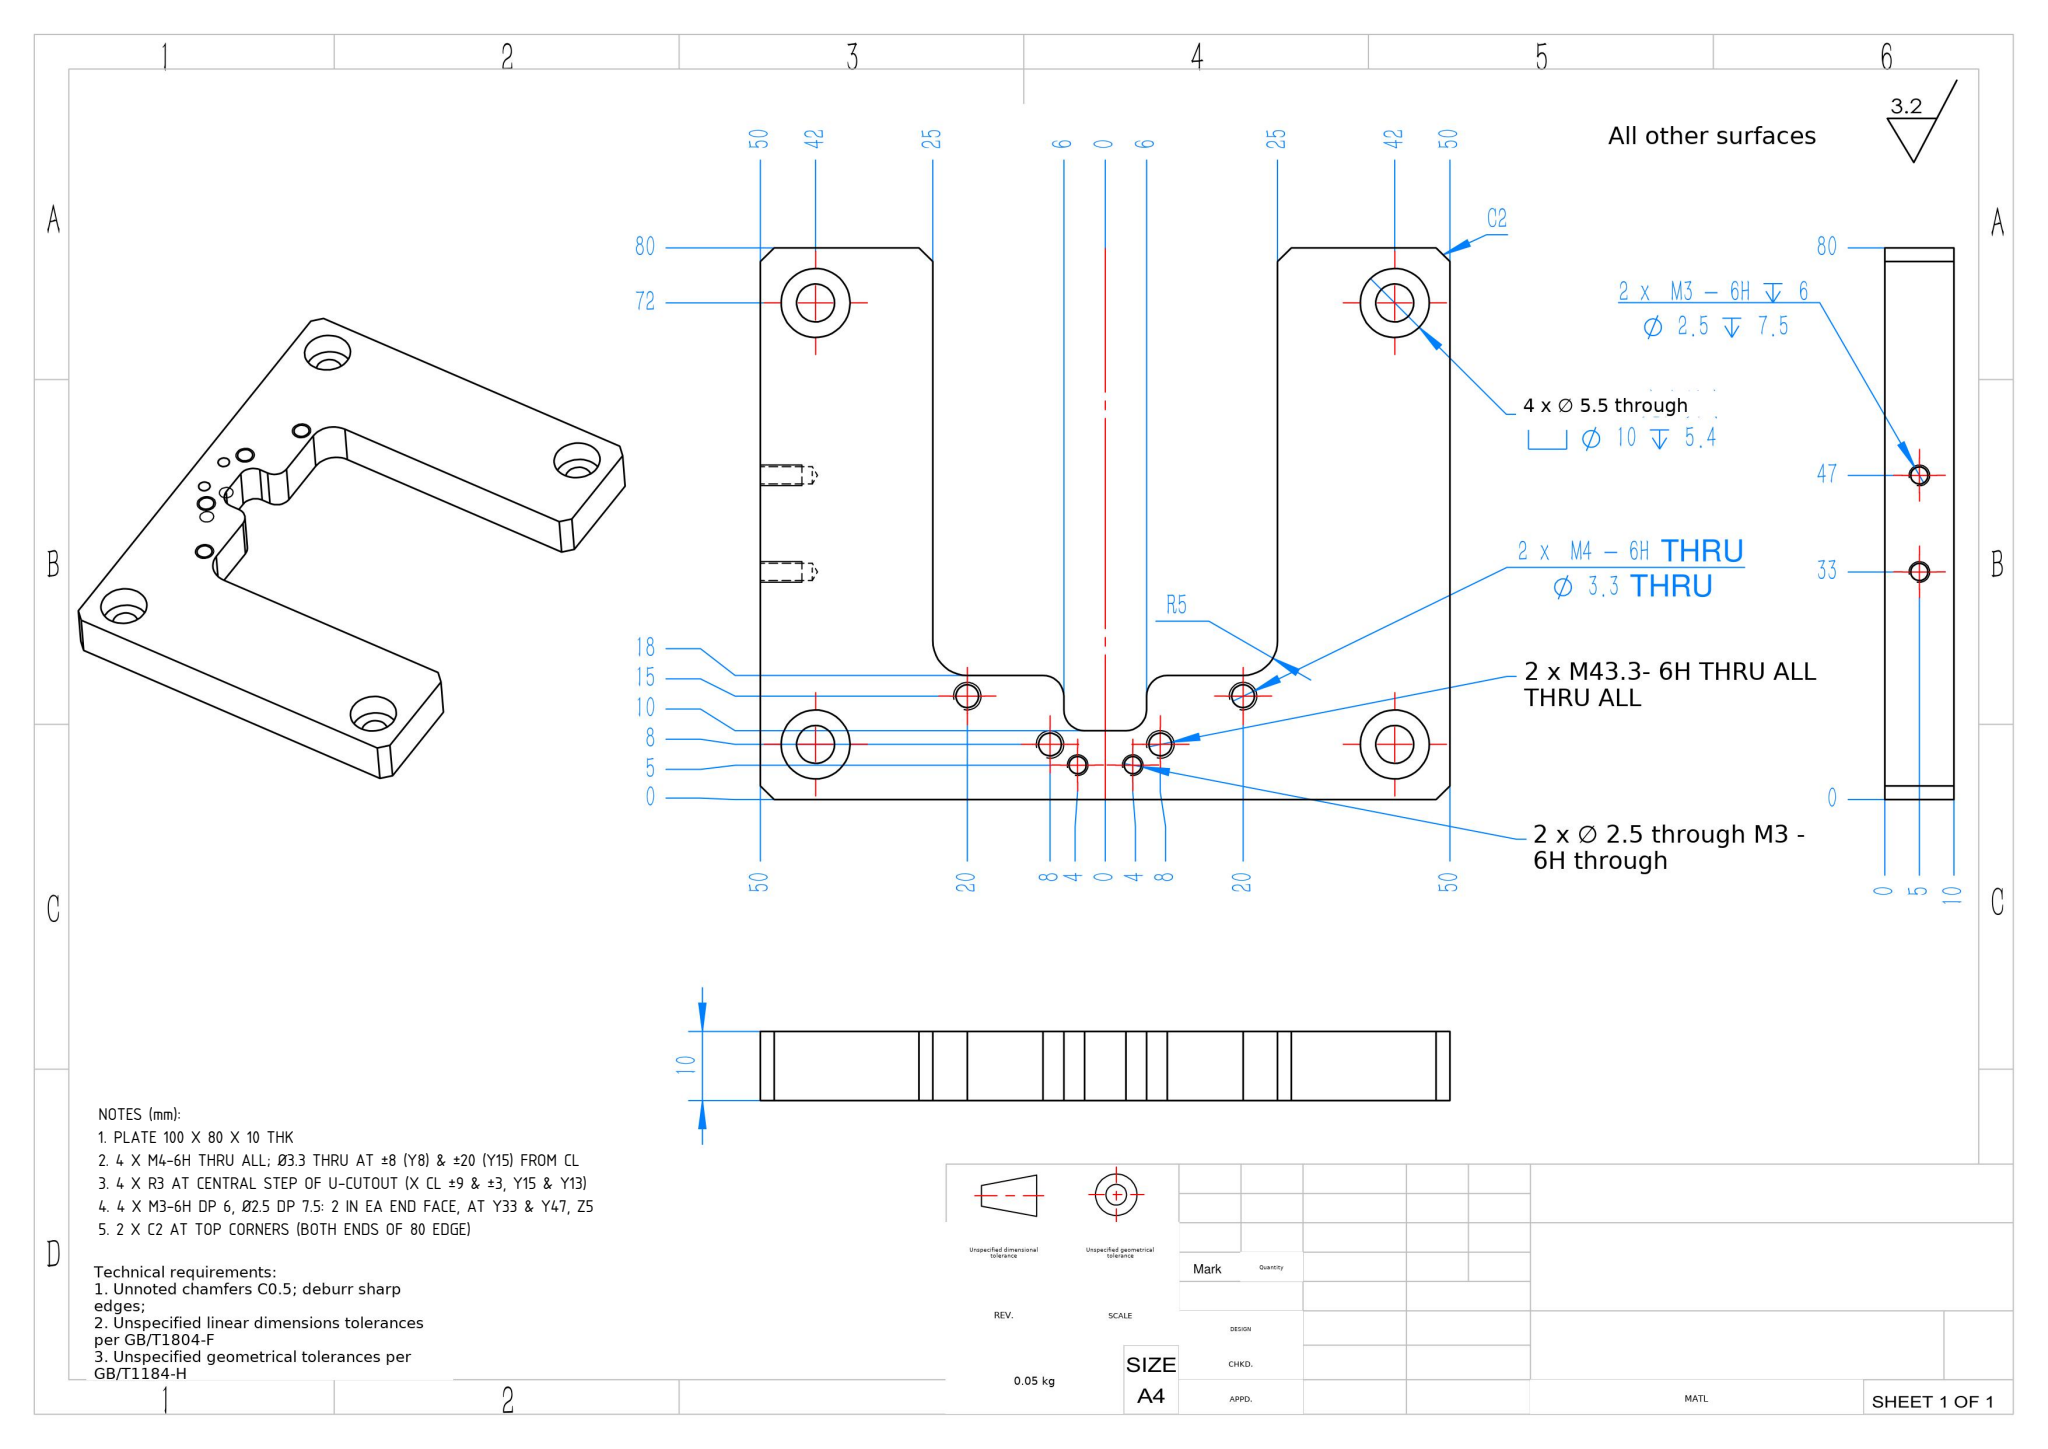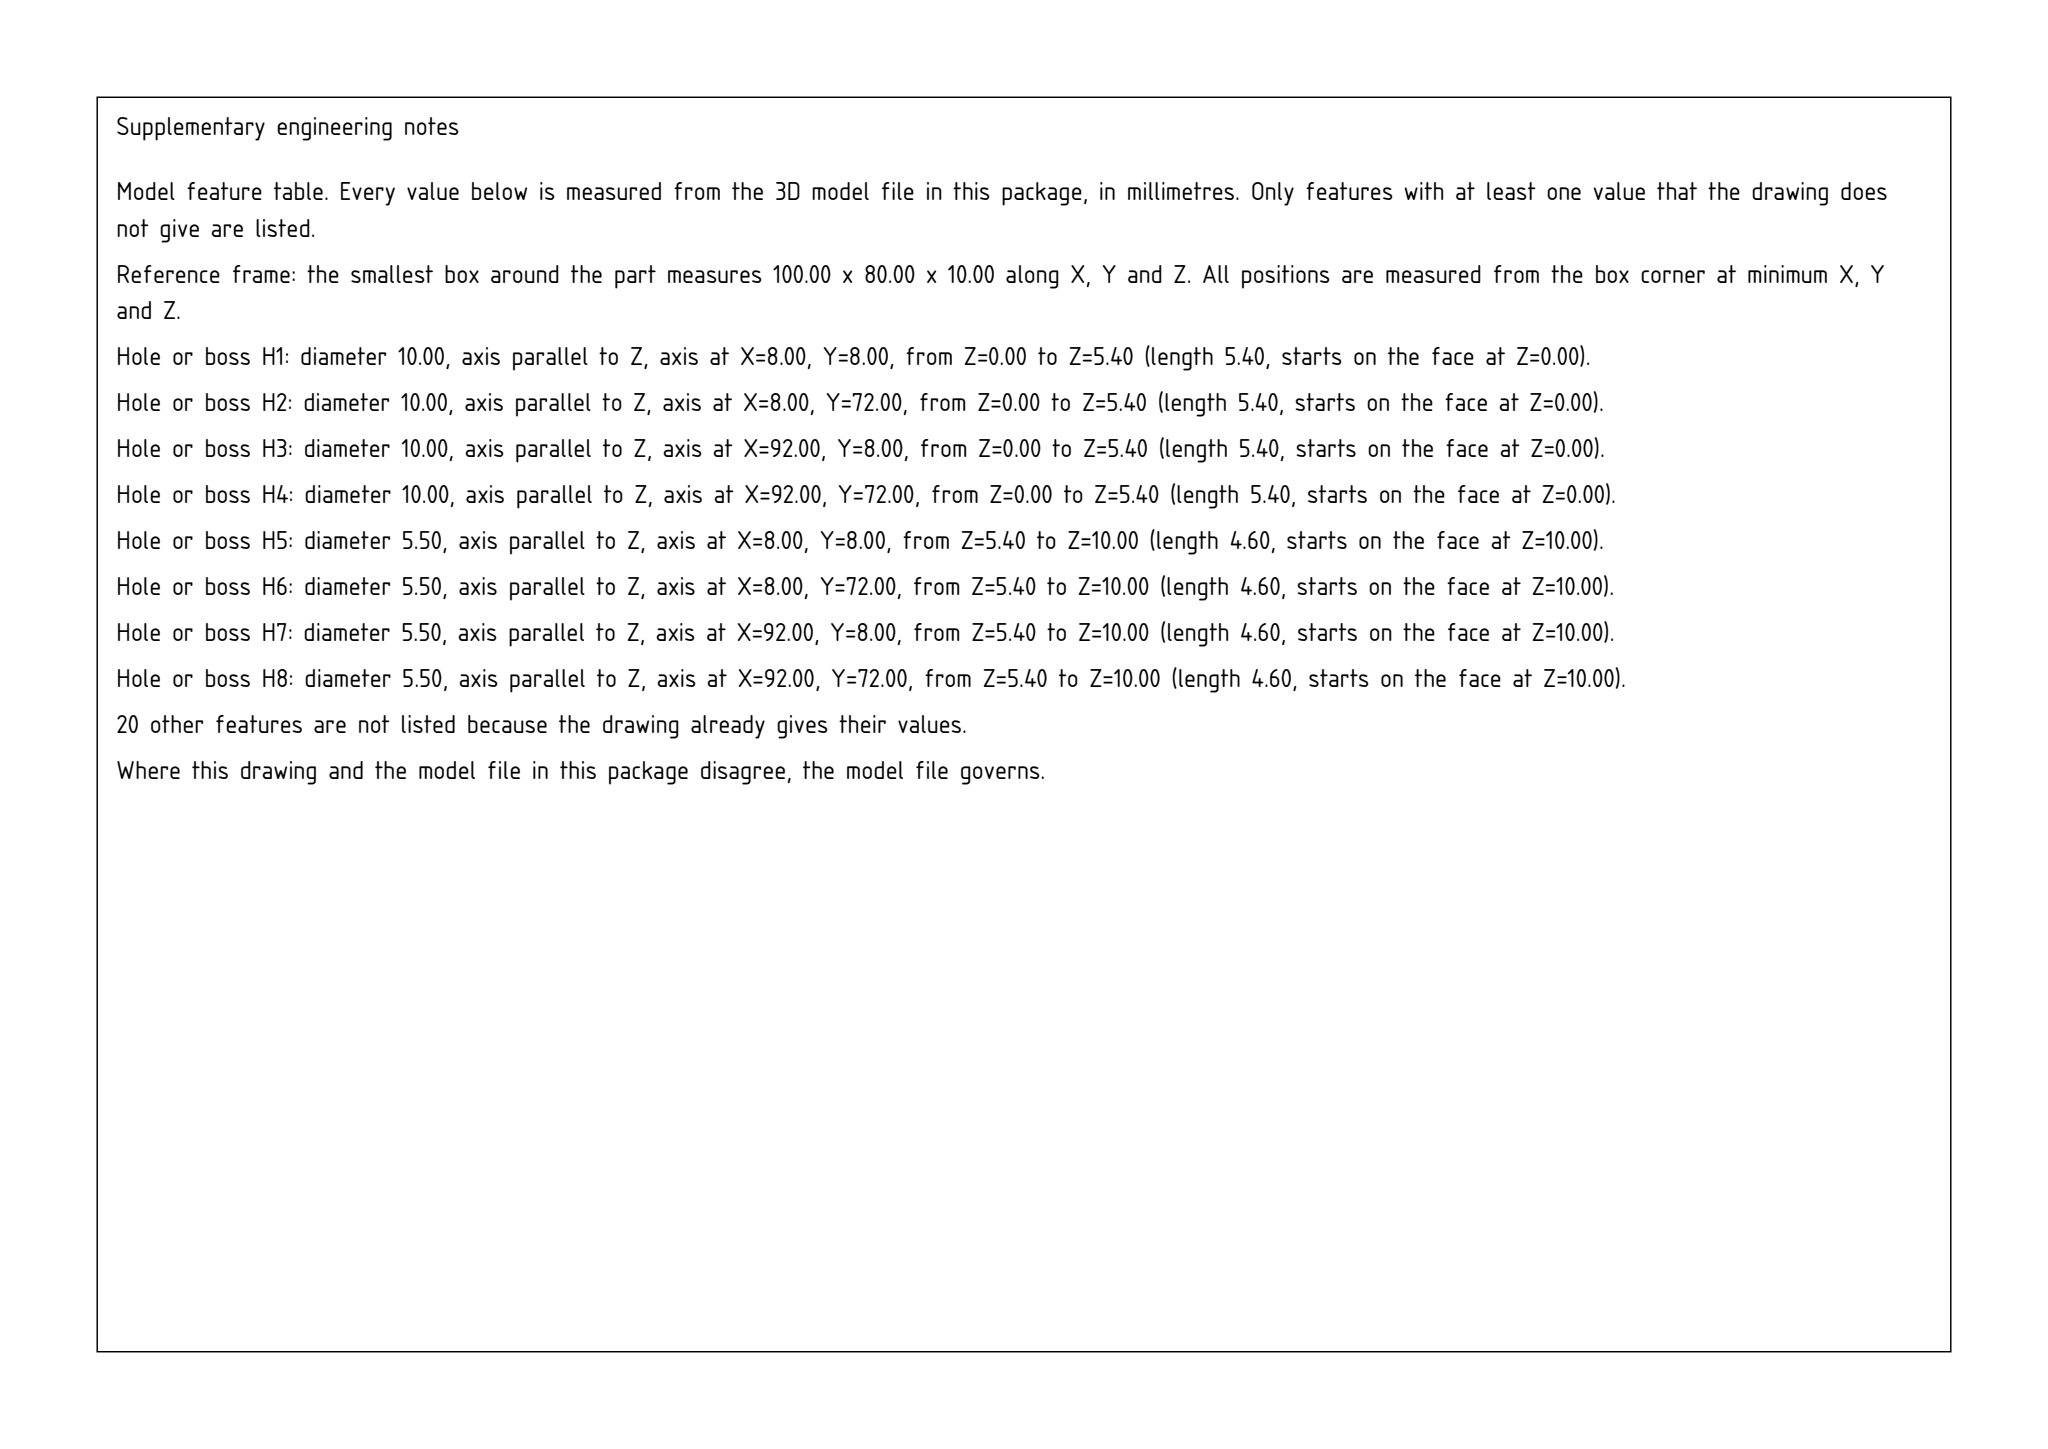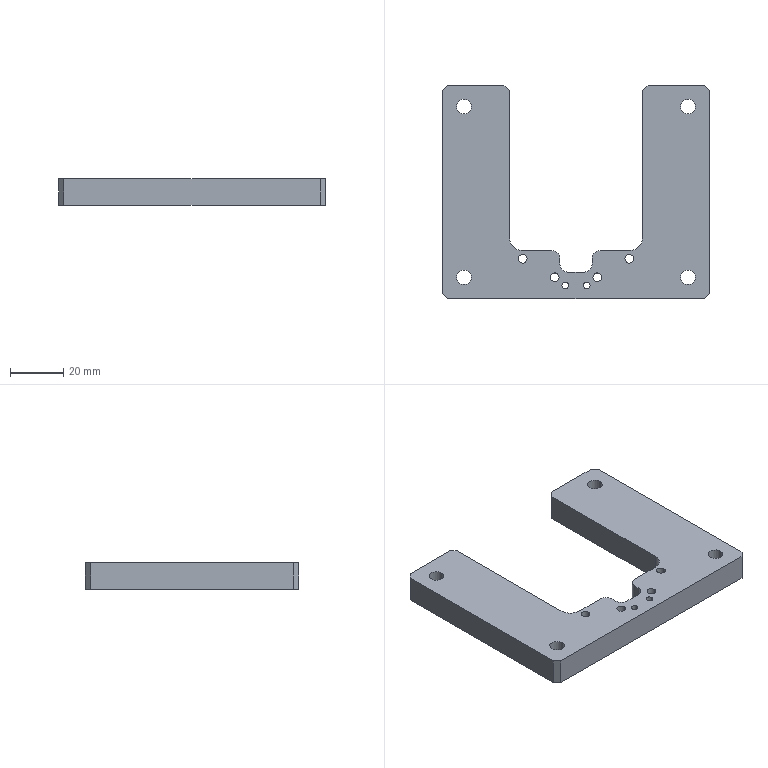Part | SolidWorks | mm | 1 solid | 66 faces | box 100 x 80 x 10 mm | volume 45377 mm3 | cylinder 38 | plane 24 | cone 4 | commonest cylinder face diameters 10 x10 2.5 x8 3.3 x8 5.5 x8 6 x4
Drawing notes:
PLATE 100 X 80 X 10 THK | from the solid: bbox_xyz 100 x 80 x 10
4 X M4-6H THRU ALL; Ø3.3 THRU AT ±8 (Y8) & ±20 (Y15) FROM CL | from the solid: Ø3.3 z-holes L10 (full thk) at (30,15),(42,8),(58,8),(70,15); CL x=50
4 X R3 AT CENTRAL STEP OF U-CUTOUT (X CL ±9 & ±3, Y15 & Y13) | from the solid: Ø6 z-cylinders at (41,15),(47,13),(53,13),(59,15) = R3; CL at X50, Y from bottom edge
4 X M3-6H DP 6, Ø2.5 DP 7.5: 2 IN EA END FACE, AT Y33 & Y47, Z5 | from the solid: Ø2.5 x-axis cylinders, len 7.5, count 2 at (y33,z5) and 2 at (y47,z5); planes x=0 and x=100
2 X C2 AT TOP CORNERS (BOTH ENDS OF 80 EDGE) | from the solid: bbox 100x80x10 with two separate faces at y=80 (axis_planes y 80: count 2) — corner cut both ends
build123d program:
from build123d import *

# Parameters (mm, degrees)
SKETCH1_W                                       = 100
SKETCH1_H                                       = 80
BOSS_EXTRUDE1_DEPTH                             = 10
M5_HEX_SOCKET_HEAD_CAP_SCREW_CBORE1_D           = 5.5
M5_HEX_SOCKET_HEAD_CAP_SCREW_CBORE1_CBORE_D     = 10
M5_HEX_SOCKET_HEAD_CAP_SCREW_CBORE1_CBORE_DEPTH = 5.4
SKETCH4_W                                       = 50
SKETCH4_H                                       = 62
CUT_EXTRUDE1_DEPTH                              = 65.807
FILLET1_R                                       = 5
CHAMFER1_SIZE                                   = 2
M4_TAPPED_HOLE1_D                               = 3.3
CUT_EXTRUDE2_DEPTH                              = 10
FILLET2_R                                       = 3
M3_TAPPED_HOLE1_D                               = 2.5
M4_TAPPED_HOLE2_D                               = 3.3
M3_TAPPED_HOLE2_D                               = 2.5
M3_TAPPED_HOLE2_DEPTH                           = 7.5
M3_TAPPED_HOLE2_TIP                             = 0.7511


with BuildPart() as part:
    # Sketch1 → Boss-Extrude1 (new body)
    with BuildSketch(Plane.XY):
        Rectangle(SKETCH1_W, SKETCH1_H)
    extrude(amount=BOSS_EXTRUDE1_DEPTH)

    # M5 Hex Socket Head Cap Screw CBORE1 (through all)
    with Locations(Plane(origin=(0, 0, 0), x_dir=(-1, 0, 0), z_dir=(0, 0, -1))):
        with Locations((-42, 32), (42, 32), (42, -32), (-42, -32)):
            CounterBoreHole(M5_HEX_SOCKET_HEAD_CAP_SCREW_CBORE1_D / 2, M5_HEX_SOCKET_HEAD_CAP_SCREW_CBORE1_CBORE_D / 2, M5_HEX_SOCKET_HEAD_CAP_SCREW_CBORE1_CBORE_DEPTH)

    # Sketch4 → Cut-Extrude1 (cut, through all)
    with BuildSketch(Plane(origin=(0, 0, 0), x_dir=(-1, 0, 0), z_dir=(0, 0, -1))):
        with Locations((0, 9)):
            Rectangle(SKETCH4_W, SKETCH4_H)
    extrude(amount=-CUT_EXTRUDE1_DEPTH, mode=Mode.SUBTRACT)

    # Fillet1
    fillet1_edges = [part.edges().sort_by_distance(p)[0] for p in [
        (25, -22, 5),
        (-25, -22, 5),
    ]]
    fillet(fillet1_edges, radius=FILLET1_R)

    # Chamfer1
    chamfer1_edges = [part.edges().sort_by_distance(p)[0] for p in [
        (25, 40, 5),
        (-25, 40, 5),
        (50, -40, 5),
        (-50, -40, 5),
        (-50, 40, 5),
        (50, 40, 5),
    ]]
    chamfer(chamfer1_edges, length=CHAMFER1_SIZE)

    # M4 Tapped Hole1 (through all)
    with Locations(Plane(origin=(0, 0, 0), x_dir=(-1, 0, 0), z_dir=(0, 0, -1))):
        with Locations((-20, -25), (20, -25)):
            Hole(M4_TAPPED_HOLE1_D / 2)

    # Sketch11 → Cut-Extrude2 (cut)
    with BuildSketch(Plane.XY.offset(10)):
        with BuildLine():
            Line((6, -22), (-6, -22))
            Line((-6, -22), (-6, -27))
            ThreePointArc((-6, -27), (-5.121, -29.121), (-3, -30))
            Line((-3, -30), (3, -30))
            ThreePointArc((3, -30), (5.121, -29.121), (6, -27))
            Line((6, -27), (6, -22))
        make_face()
    extrude(amount=-CUT_EXTRUDE2_DEPTH, mode=Mode.SUBTRACT)

    # Fillet2
    fillet2_edges = [part.edges().sort_by_distance(p)[0] for p in [
        (6, -22, 5),
        (-6, -22, 5),
    ]]
    fillet(fillet2_edges, radius=FILLET2_R)

    # M3 Tapped Hole1 (through all)
    with Locations(Plane.XY.offset(10)):
        with Locations((4, -35), (-4, -35)):
            Hole(M3_TAPPED_HOLE1_D / 2)

    # M4 Tapped Hole2 (through all)
    with Locations(Plane(origin=(0, 0, 0), x_dir=(-1, 0, 0), z_dir=(0, 0, -1))):
        with Locations((-8, -32), (8, -32)):
            Hole(M4_TAPPED_HOLE2_D / 2)

    # M3 Tapped Hole2
    with Locations(Plane(origin=(50, 0, 0), x_dir=(0, 0, -1), z_dir=(1, 0, 0))):
        with Locations((-5, 7), (-5, -7)):
            Hole(M3_TAPPED_HOLE2_D / 2, depth=M3_TAPPED_HOLE2_DEPTH)
            with Locations((0, 0, -(M3_TAPPED_HOLE2_DEPTH + M3_TAPPED_HOLE2_TIP / 2))):  # 118° drill point
                Cone(0, M3_TAPPED_HOLE2_D / 2, M3_TAPPED_HOLE2_TIP, mode=Mode.SUBTRACT)


solid = part.part